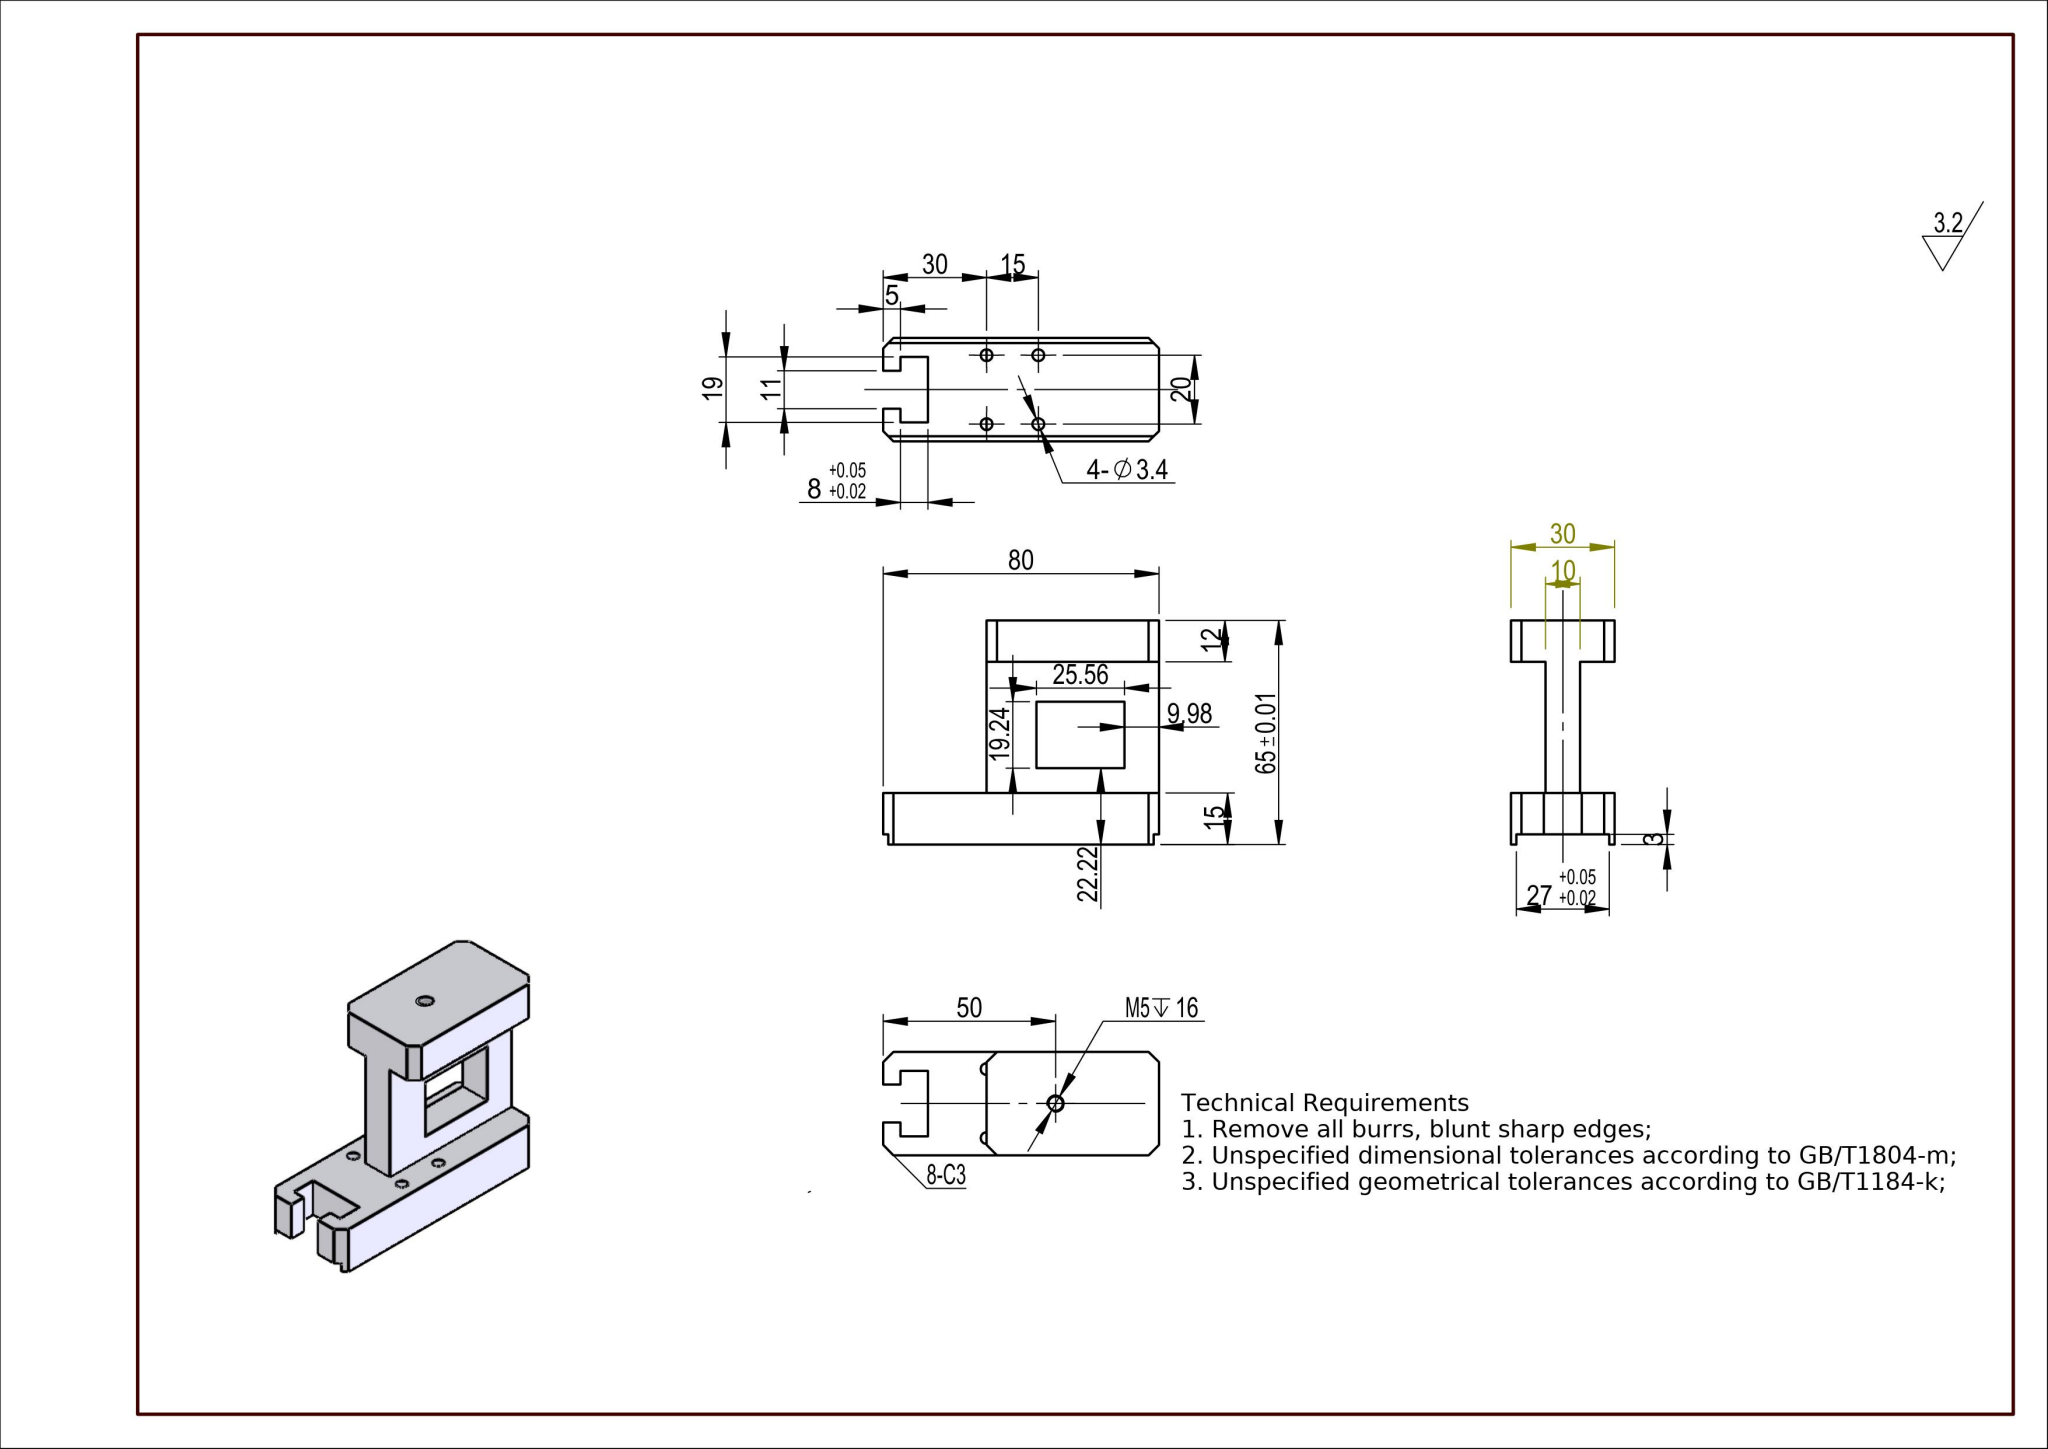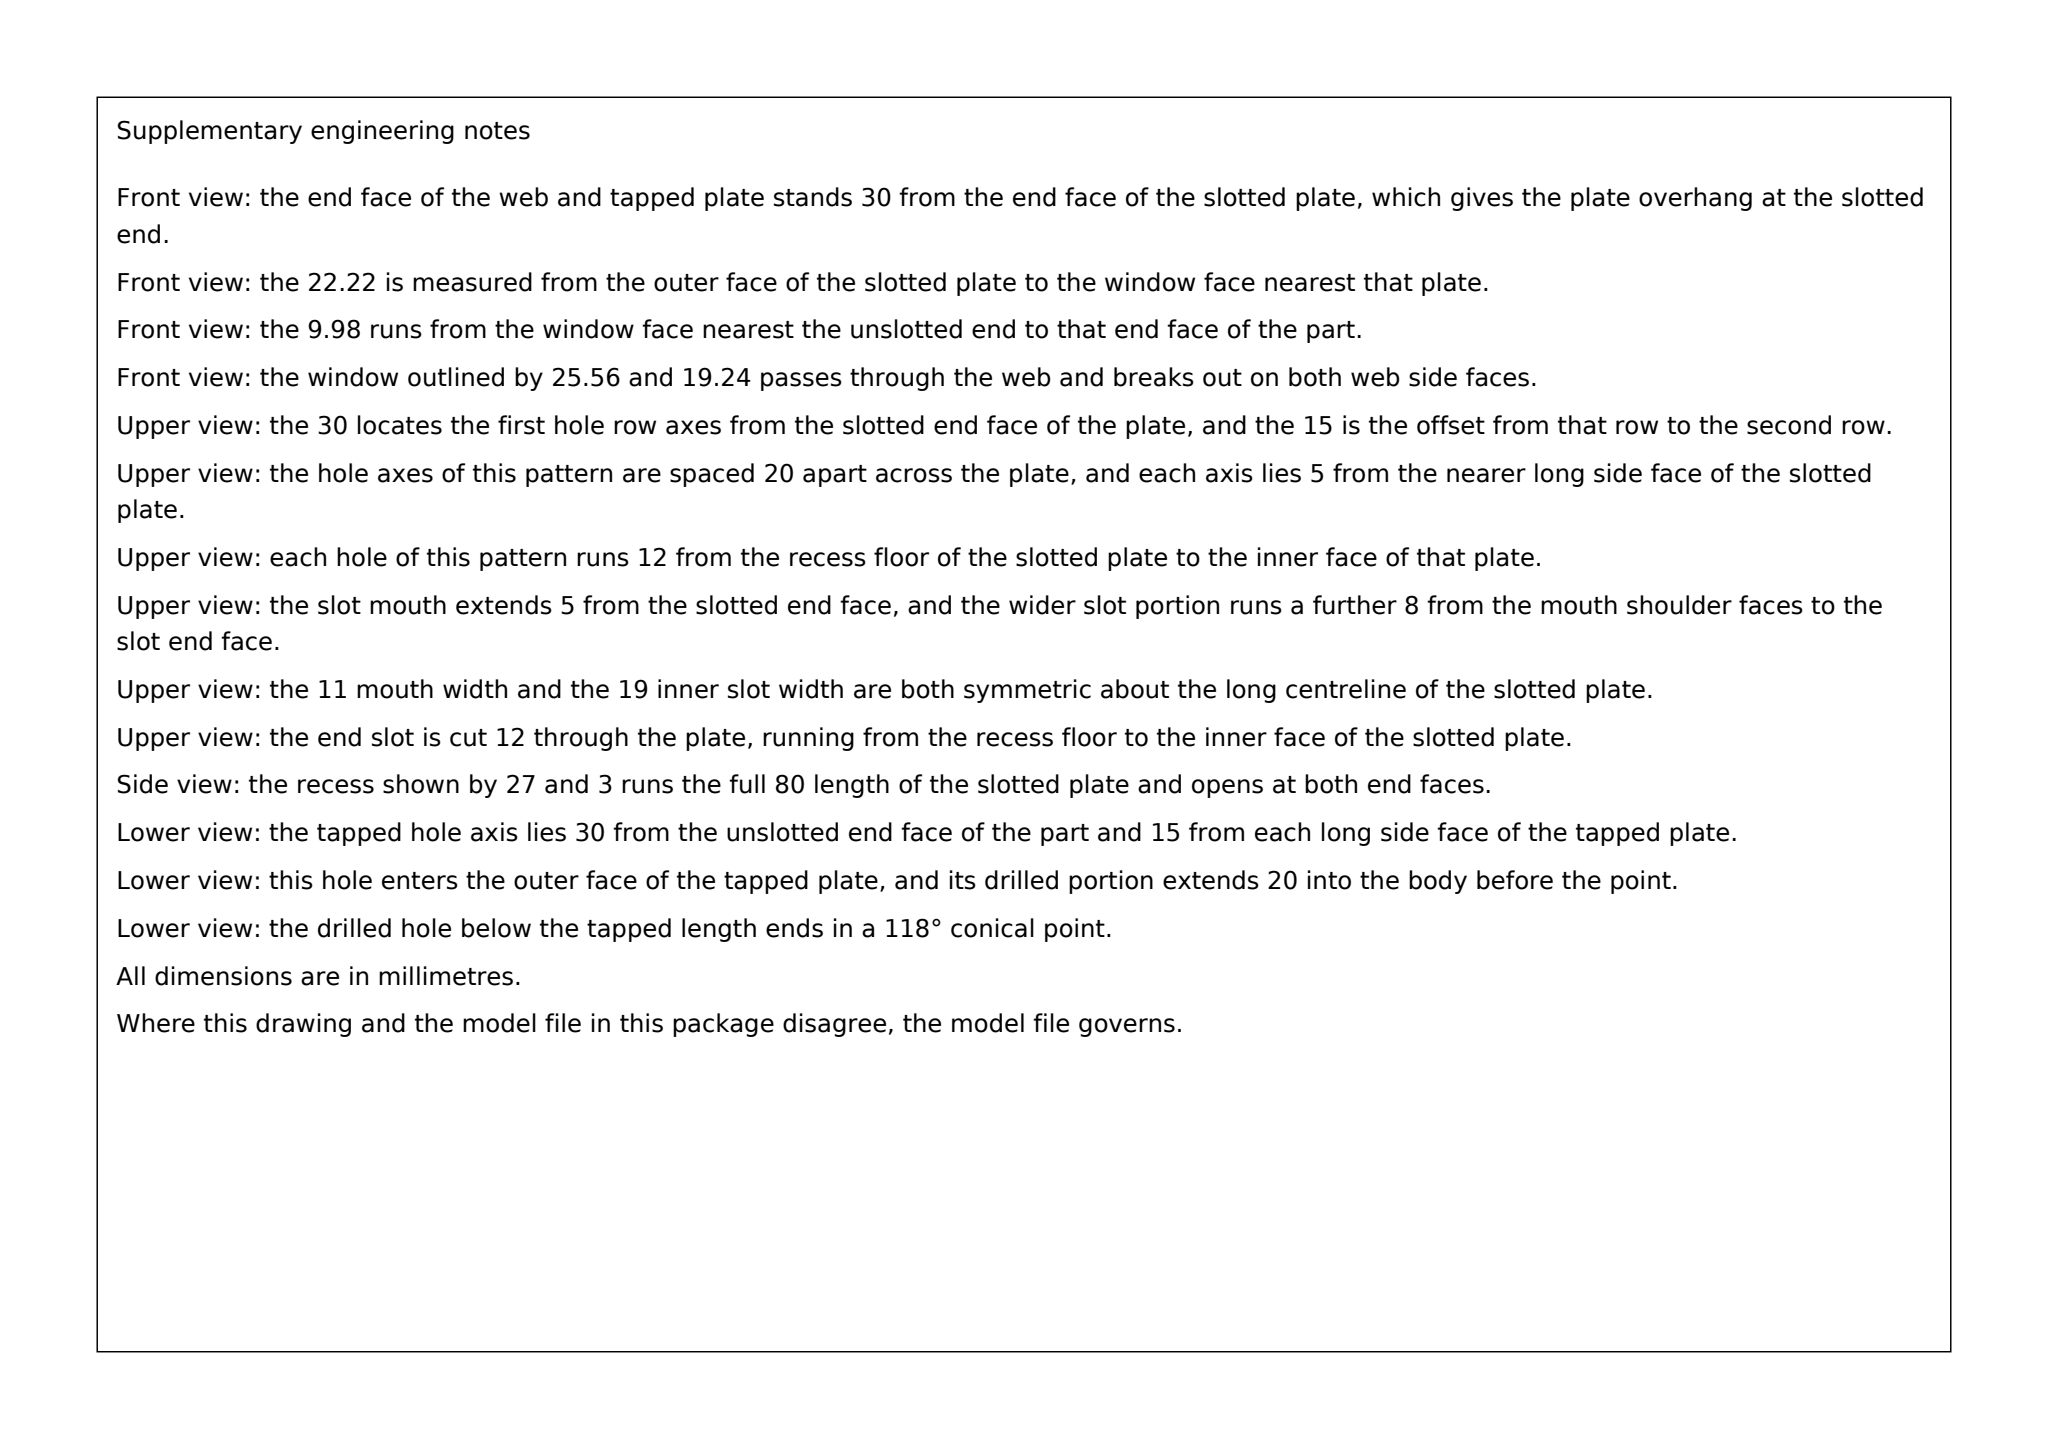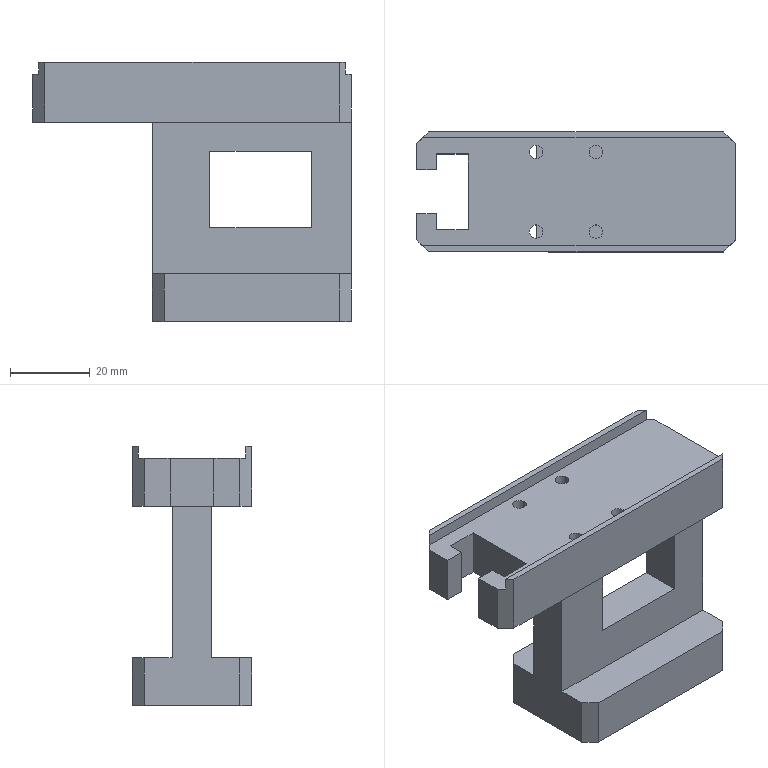Part | SolidWorks | mm | 1 solid | 50 faces | box 80 x 30 x 65 mm | volume 57928 mm3 | plane 38 | cylinder 10 | cone 2 | commonest cylinder face diameters 3.4 x8 4.2 x2
Drawing notes:
M5 TAP: Ø4.2 DRILL DP 20, 118° PT, AT X50 ON CL Y15 | from the solid: Ø4.2 z-hole at [50.0,15.0] len 20.0; cone 118° ref dia 4.2
UPRIGHT (WEB + TOP FLANGE) LEFT FACE LOCATED 30 FROM LEFT END FACE (X0); C-OPENING OVER BASE RUNS X0 TO X30 | from the solid: axis_planes[x,30.0] single vertical face bounding the upright, with bbox_xyz X=80 and base top at z=12
END T-SLOT (8 WIDE, X5 TO X13, 19 OPENING, 11 MOUTH) IS THRU THE 12 THK TOP FLANGE, Z50 TO Z62 | from the solid: T-slot faces: x=0 planes y[20.5,27.0] & y[3.0,9.5] z[50,62]; x=5 planes y[20.5,24.5] & y[5.5,9.5] z[50,62]; x=13 plane y[5.5,24.5] z[50,62]; top flange runs z50 to z62/65, base is x30-80 z0-12 with no slot
build123d program:
from build123d import *

# Parameters (mm, degrees)
SKETCH1_W                      = 80
SKETCH1_H                      = 30
BOSS_EXTRUDE1_DEPTH            = 32.5
SKETCH2_W                      = 140.082
SKETCH2_H                      = 27
CUT_EXTRUDE1_DEPTH             = 3
F_3_4_3_4_DIAMETER_HOLE1_D     = 3.4
F_3_4_3_4_DIAMETER_HOLE1_DEPTH = 20
F_3_4_3_4_DIAMETER_HOLE1_TIP   = 1.021
SKETCH5_W                      = 10
SKETCH5_H                      = 11
CUT_EXTRUDE2_DEPTH             = 78.782
SKETCH6_W                      = 8
SKETCH6_H                      = 19
CUT_EXTRUDE3_DEPTH             = 78.782
M5_TAPPED_HOLE2_D              = 4.2
M5_TAPPED_HOLE2_DEPTH          = 20
M5_TAPPED_HOLE2_TIP            = 1.262
SKETCH13_W                     = 121.156
SKETCH13_H                     = 38
CUT_EXTRUDE4_DEPTH             = 10
CUT_EXTRUDE5_REACH             = 82.889
SKETCH14_W                     = 57.856
SKETCH14_H                     = 68.267
CHAMFER1_SIZE                  = 3
SKETCH15_W                     = 25.559
SKETCH15_H                     = 19.236
CUT_EXTRUDE6_DEPTH             = 39


with BuildPart() as part:
    # Sketch1 → Boss-Extrude1 (new, symmetric)
    with BuildSketch(Plane.XY):
        Rectangle(SKETCH1_W, SKETCH1_H)
    extrude(amount=BOSS_EXTRUDE1_DEPTH, both=True)

    # Sketch2 → Cut-Extrude1 (cut)
    with BuildSketch(Plane.XY.offset(32.5)):
        Rectangle(SKETCH2_W, SKETCH2_H)
    extrude(amount=-CUT_EXTRUDE1_DEPTH, mode=Mode.SUBTRACT)

    # 3.4 _3.4_ Diameter Hole1
    with Locations(Plane(origin=(30.14, -0.2316, 29.5), x_dir=(-1, 0, 0), z_dir=(0, 0, 1))):
        with Locations((25.14, -10.232), (40.14, -10.232), (40.14, 9.768), (25.14, 9.768)):
            Hole(F_3_4_3_4_DIAMETER_HOLE1_D / 2, depth=F_3_4_3_4_DIAMETER_HOLE1_DEPTH)
            with Locations((0, 0, -(F_3_4_3_4_DIAMETER_HOLE1_DEPTH + F_3_4_3_4_DIAMETER_HOLE1_TIP / 2))):  # 118° drill point
                Cone(0, F_3_4_3_4_DIAMETER_HOLE1_D / 2, F_3_4_3_4_DIAMETER_HOLE1_TIP, mode=Mode.SUBTRACT)

    # Sketch5 → Cut-Extrude2 (cut, through all)
    with BuildSketch(Plane(origin=(0, 0, -32.5), x_dir=(-1, 0, 0), z_dir=(0, 0, -1))):
        with Locations((40, 0)):
            Rectangle(SKETCH5_W, SKETCH5_H)
    extrude(amount=-CUT_EXTRUDE2_DEPTH, mode=Mode.SUBTRACT)

    # Sketch6 → Cut-Extrude3 (cut, through all)
    with BuildSketch(Plane(origin=(0, 0, -32.5), x_dir=(-1, 0, 0), z_dir=(0, 0, -1))):
        with Locations((31, 0)):
            Rectangle(SKETCH6_W, SKETCH6_H)
    extrude(amount=-CUT_EXTRUDE3_DEPTH, mode=Mode.SUBTRACT)

    # M5 Tapped Hole2
    with Locations(Plane(origin=(0, 0, -32.5), x_dir=(-1, 0, 0), z_dir=(0, 0, -1))):
        with Locations((-10, 0)):
            Hole(M5_TAPPED_HOLE2_D / 2, depth=M5_TAPPED_HOLE2_DEPTH)
            with Locations((0, 0, -(M5_TAPPED_HOLE2_DEPTH + M5_TAPPED_HOLE2_TIP / 2))):  # 118° drill point
                Cone(0, M5_TAPPED_HOLE2_D / 2, M5_TAPPED_HOLE2_TIP, mode=Mode.SUBTRACT)

    # Sketch13 → Cut-Extrude4 (cut)
    with BuildSketch(Plane.XZ.offset(15)):
        with Locations((8.72, -1.5)):
            Rectangle(SKETCH13_W, SKETCH13_H)
    cut_extrude4 = extrude(amount=-CUT_EXTRUDE4_DEPTH, mode=Mode.SUBTRACT)

    # Mirror1: Cut-Extrude4 across plane
    add(cut_extrude4.mirror(Plane.ZX), mode=Mode.SUBTRACT)

    # Cut-Extrude5: up to this face of the body (flat: up to its plane)
    cut_extrude5_end = Plane(part.part.faces().sort_by_distance((1.689, 10.149, 17.5))[0])
    # Sketch14 → Cut-Extrude5 (cut, up to the picked face)
    with BuildSketch(Plane(origin=(-5.75, 0, -32.5), x_dir=(1, 0, 0), z_dir=(0, 0, 1)), mode=Mode.PRIVATE) as cut_extrude5_sk1:
        with Locations((-33.178, 8.581)):
            Rectangle(SKETCH14_W, SKETCH14_H)
    cut_extrude5_tool1 = split(extrude(cut_extrude5_sk1.sketch, amount=CUT_EXTRUDE5_REACH, mode=Mode.PRIVATE), bisect_by=cut_extrude5_end, keep=Keep.BOTH, mode=Mode.PRIVATE)
    add(cut_extrude5_tool1.solids().sort_by(Axis((-38.928, 8.581, -32.5), (0, 0, 1)))[0], mode=Mode.SUBTRACT)

    # Chamfer1
    chamfer1_edges = [part.edges().sort_by_distance(p)[0] for p in [
        (-40, 15, 25),
        (-40, -15, 25),
        (40, -15, 25),
        (40, -15, -26.5),
        (40, 15, 25),
        (40, 15, -26.5),
        (-10, 15, -26.5),
        (-10, -15, -26.5),
    ]]
    chamfer(chamfer1_edges, length=CHAMFER1_SIZE)

    # Sketch15 → Cut-Extrude6 (cut)
    with BuildSketch(Plane.XZ.offset(5)):
        with Locations((17.239, 0.6656)):
            Rectangle(SKETCH15_W, SKETCH15_H)
    extrude(amount=-CUT_EXTRUDE6_DEPTH, mode=Mode.SUBTRACT)


solid = part.part